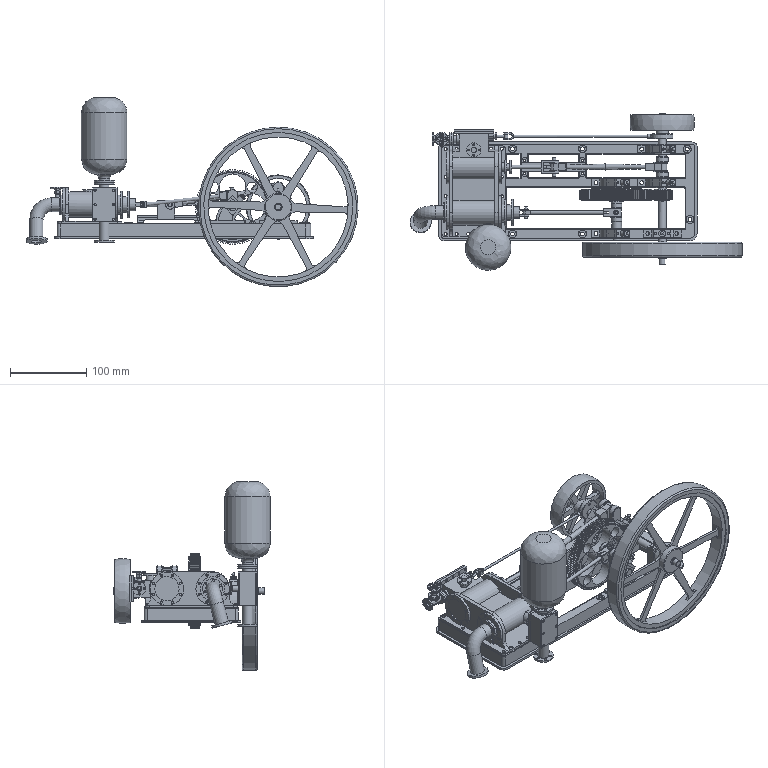Assembly | NX | mm | 86 component files | 86 solids | 2631 faces | box 436.98 x 206 x 248.97 mm | volume 711241 mm3 | cylinder 1021 | plane 907 | other 480 | spline 134 | torus 66 | cone 18 | sphere 5 | commonest cylinder face diameters 3 x200 2 x150 93.5 x96 5 x87 4 x55 2.5 x51 10 x47 6 x39
Bill of materials:
unnamed part 1 | 1 |  | Long slender cylindrical pin with a countersunk-style conical head, a short larger-diameter shoulder section below the head, then a long smaller-diameter plain shank ending in a flat end.
unnamed part 2 | 1 |  | Clevis/fork block: rectangular solid body with a rectangular slot open at one end, forming two parallel lugs with rounded ends and aligned through-holes; a smaller through-hole passes through the body at the base of the slot.
unnamed part 3 | 1 |  | Stepped annular flange body: a larger-diameter disc and a smaller-diameter disc joined by a cylindrical hub, all sharing a large central bore; both discs have rings of axial bolt holes (8 visible in face view).
unnamed part 4 | 1 |  | Hollow cylindrical tube, open at one end, with the other end closed by a rounded/conical taper ending in a short small-diameter neck with a central through-hole.
unnamed part 5 | 1 |  | Plain flat annular ring (washer- or spacer-like) with a centred circular through-hole and moderate thickness.
unnamed part 6 | 1 |  | Thick cylindrical sleeve/bushing with a large concentric through-bore and a relatively thin wall compared with the similar ring part.
unnamed part 7 | 1 |  | Long round rod with a rounded eye end at one end (transverse through-hole) and a square block at the other end with a small square hole and a slot.
unnamed part 8 | 1 |  | Very long slender round rod with a small clevis fork at one end: two parallel lugs with aligned cross-holes; the opposite end is plain.
unnamed part 9 | 5 |  | Rectangular flat plate (block) with one large central through-hole and two smaller through-holes, one near each end, all in a line along the long axis.
unnamed part 10 | 4 |  | Angled bracket: a flat base strip with a through-hole at each end, and a raised web rising at about 45 degrees into a U-shaped fork with two parallel tabs, each with a through-hole; fillets blend the web into the base.
unnamed part 11 | 1 |  | Housing/frame: a rectangular base plate with perimeter holes, two upright end plates with rounded tops, each with two large bores and surrounding small hole patterns, joined by two parallel cylindrical shells; a small cylindrical boss with a bore projects from one shell near one end plate.
unnamed part 12 | 1 |  | Flanged tee-shaped body: a barrel-shaped, bulging central body with a circular flange at each end and a third circular flange on a short branch on top; each flange has four bolt holes and a central bore.
unnamed part 13 | 1 |  | Short hollow cylinder with one step: a wider ring section at one end and a slightly smaller-diameter section at the other, with a plain through bore. Looks like a flanged bushing or sleeve.
unnamed part 14 | 1 |  | Bracket with a flat rectangular base plate and two parallel rectangular uprights, forming a U-shaped fork in the front profile. The base has one through hole at each end, each upright has a small hole in its top face, and there are fillets where the uprights meet the base.
unnamed part 15 | 1 |  | Thin-walled circular ring or band with one short solid cylindrical stub sticking out radially from its outer surface. The stub has a small fillet where it joins the ring.
unnamed part 16 | 1 |  | Long, slender cylindrical rod. At one end it joins, at right angles, a short hollow cylindrical boss or eye with a through bore, whose axis is perpendicular to the rod.
unnamed part 17 | 1 |  | Thin flat ring with a small step: a slightly larger outer diameter on one face and a slightly smaller one on the other. It has a large central bore relative to its outer diameter.
unnamed part 18 | 1 |  | Straight-tooth spur gear with about 24 external teeth, a central through bore with a single rectangular keyway, and a raised hub face or shoulder on each side.
unnamed part 19 | 1 |  | Solid stepped cylindrical pin or shaft: a larger-diameter central body with smaller-diameter coaxial journals at both ends.
unnamed part 20 | 1 |  | Prismatic block with angled (chamfered) faces on one side and a rounded-end U-slot cut in from that side. It has a stepped profile (a narrower raised portion on a wider base) and a rectangular recess or pocket visible in one face of the isometric view.
unnamed part 21 | 1 |  | Block with a through bore. In the end profile one side is a rounded semicircle and the other side tapers to flat faces, giving a teardrop or D shape. Thin raised lips or flanges at both axial ends border a slightly recessed middle band.
unnamed part 22 | 1 |  | Spoked wheel with six straight spokes joining a central hub to an outer rim. The hub has a small central through hole and the rim has a slightly crowned outer surface.
unnamed part 23 | 1 |  | Thin circular disc with rounded edges, pierced by four large circular holes evenly spaced around a smaller central hole.
unnamed part 24 | 5 |  | Ball stud: a spherical ball on a short narrowed neck, standing on a cylindrical disc base. The base appears stepped, with a smaller-diameter boss or section on the side opposite the ball.
unnamed part 25 | 1 |  | Flanged cylindrical bushing: a short cylindrical shank joined to a larger-diameter cylindrical flange, with a plain through bore on the common axis.
unnamed part 26 | 1 |  | Thin-walled plain ring: short hollow cylinder with a large bore and a narrow radial wall.
unnamed part 27 | 1 |  | Grooved disc/pulley-like wheel: solid cylindrical disc with one rectangular circumferential groove at mid-width and a small central through bore.
unnamed part 28 | 1 |  | Spur gear with straight external teeth and a web pierced by lightening holes: four large and four small circular cutouts arranged around a central bore that has a keyway notch.
unnamed part 29 | 1 |  | Plain flat ring/washer-like annulus with a moderate radial wall, thicker relative to its diameter than the other thin ring.
unnamed part 30 | 1 |  | Stepped solid cylindrical shaft/pin: a longer central section of larger diameter with a shorter, smaller-diameter journal at each end.
unnamed part 31 | 1 |  | Thin flat circular disc/washer with a small central through hole.
unnamed part 32 | 1 |  | Flanged hub/flange mount: a round flange with four through holes on a bolt circle, a coaxial cylindrical boss on one side, and a central through bore.
unnamed part 33 | 1 |  | Elongated mounting bracket/strap: a long rectangular bar with a T-shaped end profile, supported at each end by filleted posts down to flat foot lugs. Each end has two rounded-end tabs, each with a through hole (four holes in total).
unnamed part 34 | 1 |  | Clamp/bearing-block-like body: a block with one flat, slightly tapered mounting side and one semicircular rounded side. It has a large through bore, a raised lip or rim at each axial end, and a small radial hole through the top into the bore.
unnamed part 35 | 1 |  | Flat rectangular plate with six round through holes, three evenly spaced along each long edge.
unnamed part 36 | 1 |  | Stepped solid cylindrical shaft with four coaxial diameters that get smaller from a large base section to a slender tip section.
unnamed part 37 | 1 |  | Single-throw crank-shaped shaft: two coaxial cylindrical end shafts joined by two parallel obround webs and an offset cylindrical pin between them.
unnamed part 38 | 1 |  | Circular flat flange plate with a raised cylindrical hub in the center, a central through bore, and four through holes evenly spaced on a bolt circle.
unnamed part 39 | 5 |  | Square block with rounded corners and a large round through bore along its axis. Square end flanges stand slightly proud of an inset middle body.
unnamed part 40 | 1 |  | Round drum with a rim flange at each end, forming a shallow groove between them, plus a smaller cylindrical hub on one side. The hub's through bore is off-center from the drum, and a small through hole sits on the opposite side of the face.
unnamed part 41 | 1 |  | Flat circular flange ring with a central bore, eight through holes evenly spaced on a bolt circle, and a raised annular face around the bore.
unnamed part 42 | 1 |  | Hexagonal prism with a plain cylindrical through hole in the center.
unnamed part 43 | 1 |  | 90-degree bent tube with a flange at each end. One flange has six bolt holes; the other is a plain annular flange with no visible holes.
unnamed part 44 | 1 |  | D-shaped block, rounded at one end and flat at the other, with a large round through bore. Thin lips at both ends stand slightly proud of the middle body.
unnamed part 45 | 1 |  | Flanged bushing: a circular flange with four bolt holes, a cylindrical shank on one side, and a central through bore.
unnamed part 46 | 1 |  | Plain flat annular ring (washer shape) with a central round hole.
unnamed part 47 | 1 |  | Short tubular neck joined to a circular flange with six evenly spaced bolt holes and a central through bore.
unnamed part 48 | 1 |  | Solid circular disc (blind-flange shape) with eight evenly spaced bolt holes and a raised circular face on one side; there is no central bore.
unnamed part 49 | 1 |  | Flanged cylindrical hub: a circular flange with four through holes, a cylindrical hub with a raised collar ring partway along it, and a central through bore.
unnamed part 50 | 1 |  | Solid rectangular block with one cylindrical through hole passing straight through between two opposite faces.
unnamed part 51 | 5 |  | Short hollow cylindrical sleeve (bushing-like tube) with a stepped outer diameter: a reduced-diameter band at one end.
unnamed part 52 | 1 |  | Slender rod with a square block at each end. The faceted shaft tapers from a thicker middle toward both ends.
unnamed part 53 | 1 |  | Vertical housing made of a rectangular box with open, bolt-holed rims on two sides, plus pipe stubs ending in circular bolted flanges top and bottom.
unnamed part 54 | 1 |  | Rectangular mounting plate with six perimeter holes and a central hole. A cylindrical pipe stub projects perpendicular from one face and ends in a circular flange.
unnamed part 55 | 1 |  | Diamond-shaped (two-lobe) flange with rounded ends, a hole in each lobe, a larger central through hole, and a cylindrical boss on one side.
unnamed part 56 | 1 |  | Thin strip bent into a U (hairpin) shape. Each leg has a slot open at its end, and a short hollow cylindrical boss stands on the outer face near the bend.
unnamed part 57 | 1 |  | Long straight round pin/shaft with a reduced-diameter step at each end.
unnamed part 58 | 1 |  | Box-like bracket with a channel-shaped body, two round-ended lugs with coaxial through holes, an elongated slot in one face, a hole in another face, and hooked/stepped feet at the bottom.
unnamed part 59 | 1 |  | Long rectangular frame plate with rounded corners, divided by webs into six rectangular through openings. It has many small holes around the perimeter and on the webs, several raised or counterbored hole bosses, and a stepped lip around the base.
unnamed part 60 | 1 |  | Spoked wheel: a circular rim joined by six straight spokes to a central hub with a small central bore.
unnamed part 61 | 1 |  | Round flange part: a large flat circular disc with a ring of 8 through-holes near its edge and a central bore. A short shallow raised step is on one face. On the other face, a cylindrical neck sticks out and ends in a smaller circular flange with its own ring of small holes around the central bore.
unnamed part 62 | 1 |  | Cup-shaped wheel: a thin-walled cylindrical rim with two grooves running around its outside. A web sits inside the rim, recessed from one face, with a central hole and six large round lightening holes evenly spaced around it.
unnamed part 63 | 1 |  | Plain flat ring (annulus) with a large central through-hole and parallel flat faces, shaped like a washer.
unnamed part 64 | 1 |  | Capsule-shaped closed body: a cylinder with rounded, dome-like ends. At one end, a short narrow neck flares into a small circular flange with several small holes.
unnamed part 65 | 1 |  | Machined block bracket: a flat rectangular mounting plate with two rows of 5 through-holes, joined at a right angle to a block-shaped body. The body has a flat top with a counterbored hole, ledges/rails along its long sides, a concave curved cutout at the end away from the plate, elongated slots through the body, and a boss with a bore and small holes next to the plate.
unnamed part 66 | 1 |  | Single-throw crank-type shaft: a long stepped cylindrical shaft with two parallel obround (rounded-end) webs near one end, joined by an offset cylindrical pin. Several short diameter steps run along the shaft, with shallow slot-like features that may be keyways.
unnamed part 67 | 1 |  | Flat rectangular plate of constant thickness with 14 round through-holes spaced along its edges: 5 along each long edge (including the corners) and 2 more along each short edge.
Mates:
1. fix | base 1 component
2. concentric | base 1 edge | support_stand 1 edge
3. parallel | support_stand 1 face | base 1 face
4. concentric | base 1 edge | inclined_frame 4 arc
5. parallel | inclined_frame 4 face | base 1 face
6. concentric | inclined_frame 4 edge | inclined_frame_top_plate 5 arc
7. parallel | inclined_frame_top_plate 5 face | inclined_frame 4 face
8. center | inclined_frame 4 face | inclined_frame 4 face | filler_block 5 face | filler_block 5 face
9. center | filler_block 5 face | filler_block 5 face | inclined_frame 4 face | inclined_frame 4 face
10. touch align | filler_block 5 face | inclined_frame 4 face
11. concentric | base 1 edge | inclined_frame 3 arc
12. parallel | inclined_frame 3 face | base 1 face
13. concentric | base 1 edge | inclined_frame 2 arc
14. parallel | inclined_frame 2 face | base 1 face
15. concentric | base 1 edge | inclined_frame 1 arc
16. parallel | inclined_frame 1 face | base 1 face
17. concentric | inclined_frame 3 edge | inclined_frame_top_plate 4 arc
18. parallel | inclined_frame_top_plate 4 face | inclined_frame 3 face
19. concentric | inclined_frame 2 edge | inclined_frame_top_plate 3 arc
20. parallel | inclined_frame_top_plate 3 face | inclined_frame 2 face
21. concentric | inclined_frame 1 edge | inclined_frame_top_plate 2 arc
22. parallel | inclined_frame_top_plate 2 face | inclined_frame 1 face
23. center | filler_block 4 face | filler_block 4 face | inclined_frame 3 face | inclined_frame 3 face
24. center | filler_block 4 face | filler_block 4 face | inclined_frame 3 face | inclined_frame 3 face
25. touch align | filler_block 4 face | inclined_frame_top_plate 4 face
26. center | filler_block 3 face | filler_block 3 face | inclined_frame 2 face | inclined_frame_top_plate 3 face
27. center | filler_block 3 face | filler_block 3 face | inclined_frame 2 face | inclined_frame 2 face
28. touch align | filler_block 3 face | inclined_frame 2 face
29. center | filler_block 2 face | filler_block 2 face | inclined_frame 1 face | inclined_frame_top_plate 2 face
30. center | filler_block 2 face | filler_block 2 face | inclined_frame 1 face | inclined_frame 1 face
31. touch align | filler_block 2 face | inclined_frame 1 face
32. touch align | base 1 face | piston_cyl_body 1 face
33. center | piston_cyl_body 1 face | piston_cyl_body 1 face | base 1 face | base 1 face
34. touch align | piston_cyl_body 1 face | ext_cylinder_body 1 face
35. center | ext_cylinder_body 1 face | ext_cylinder_body 1 face | piston_cyl_body 1 face | piston_cyl_body 1 face
36. concentric | ext_cylinder_body 1 edge | ext_end_plate 1 arc
37. parallel | ext_end_plate 1 face | ext_cylinder_body 1 face
38. concentric | piston_cyl_body 1 edge | air_cylinder_conn_plate 1 arc
39. parallel | air_cylinder_conn_plate 1 face | base 1 face
40. concentric | air_cylinder_conn_plate 1 edge | water_tank_cyl_body 1 edge
41. parallel | water_tank_cyl_body 1 face | air_cylinder_conn_plate 1 face
42. concentric | water_cyl_tank_end_plate 1 arc | water_tank_cyl_body 1 edge
43. parallel | water_cyl_tank_end_plate 1 face | water_tank_cyl_body 1 face
44. concentric | water_tank_cyl_body 1 edge | water_chamber 1 arc
45. concentric | water_chamber 1 edge | water_tank_cyl_body 1 edge
46. touch align | crankshaft 1 face | filler_block 2 face
47. center | crankshaft 1 face | crankshaft 1 face | piston_cyl_body 1 face
48. touch align | filler_block 1 face | crankshaft 1 face
49. center | filler_block 1 face | filler_block 1 face | base 1 face | base 1 face
50. parallel | filler_block 1 face | base 1 face
51. touch align | filler_block 1 face | inclined_frame_top_plate 1 face
52. center | inclined_frame_top_plate 1 face | inclined_frame_top_plate 1 face | filler_block 1 face | filler_block 1 face
53. concentric | upright_frame 1 arc | inclined_frame_top_plate 1 edge
54. parallel | upright_frame 1 face | inclined_frame_top_plate 1 face
55. touch align | big_flywheel 1 face | crankshaft 1 face
56. distance | big_flywheel 1 face | base 1 face
57. touch align | small_gear 1 face | crankshaft 1 face
58. touch align | crankshaft_2 1 face | filler_block 5 face
59. center | crankshaft_2 1 face | crankshaft_2 1 face | piston_cyl_body 1 face
60. touch align | big_gear 1 face | crankshaft_2 1 face
61. parallel | crankshaft_2 1 face | big_gear 1 face
62. center | big_gear 1 face | big_gear 1 face | filler_block 4 face | crankshaft_2 1 face
63. center | small_gear 1 face | small_gear 1 face | big_gear 1 face | big_gear 1 face
64. concentric | washer 1 arc | big_gear 1 edge
65. touch align | link_1 1 face | big_conn_block 1 face
66. center | link_1 1 face | link_1 1 face | big_conn_block 1 face | big_conn_block 1 face
67. center | link_1 1 face | link_1 1 face | big_conn_block 1 face | big_conn_block 1 face
68. touch align | link_1 1 face | small_conn_block 1 face
69. center | small_conn_block 1 face | small_conn_block 1 face | link_1 1 face | link_1 1 face
70. center | small_conn_block 1 face | small_conn_block 1 face | link_1 1 face | link_1 1 face
71. touch align | big_conn_block 1 face | crankshaft 1 face
72. center | big_conn_block 1 face | big_conn_block 1 face | piston_cyl_body 1 face
73. concentric | piston_ring 1 arc | piston 1 edge
74. concentric | link_2 1 edge | piston 1 arc
75. touch align | link_2 1 face | piston_cyl_body 1 face
76. distance | piston_cyl_body 1 face | base 1 face
77. concentric | link_slider 1 arc | link_2 1 edge
78. touch align | small_conn_block 1 face | link_slider 1 face
79. touch align | link_pin 1 face | link_slider 1 face
80. center | link_pin 1 face | link_pin 1 face | link_slider 1 face | link_slider 1 face
81. center | link_3_large_block 1 face | link_3_large_block 1 face | link_3 1 face | link_3 1 face
82. touch align | link_3_large_block 1 face | link_3 1 face
83. center | link_3_large_block 1 face | link_3_large_block 1 face | link_3 1 face | link_3 1 face
84. touch align | link_3_large_block 1 face | crankshaft_2 1 face
85. center | link_3_large_block 1 face | link_3_large_block 1 face | crankshaft_2 1 face | crankshaft_2 1 face
86. concentric | link_3_large_ring 1 edge | link_3_large_block 1 edge
87. parallel | link_3 1 face | link_3_large_ring 1 face
88. concentric | round_plate 1 edge | link_4 1 edge
89. concentric | int_pipe_flywheel 1 edge | round_plate 1 arc
90. concentric | lumen 1 arc | int_pipe_flywheel 1 arc
91. concentric | link_4_block 1 edge | link_4 1 edge
92. touch align | link_4_block 1 face | link_3 1 face
93. center | link_4_block 1 face | link_4_block 1 face | link_3 1 face | link_3 1 face
94. touch align | lumen 1 face | piston_cyl_body 1 face
95. touch align | link_4_pin 1 face | link_4_block 1 face
96. center | link_4_pin 1 face | link_4_pin 1 face | link_4_block 1 face | link_4_block 1 face
97. concentric | link_5 1 arc | link_5_ring 1 edge
98. parallel | link_5 1 face | link_5_ring 1 face
99. touch align | eccentric_cam 1 face | link_5_ring 1 face
100. center | eccentric_cam 1 face | eccentric_cam 1 face | link_5_ring 1 face | link_5_ring 1 face
101. touch align | eccentric_cam 1 face | crankshaft 1 face
102. center | eccentric_cam 1 face | eccentric_cam 1 face | ext_cylinder_body 1 face
103. touch align | link_6 1 face | link_5 1 face
104. center | link_5 1 face | link_5 1 face | link_6 1 face | link_6 1 face
105. touch align | link_6 1 face | ext_cylinder_body 1 face
106. concentric | piston_cyl_body 1 edge | end_cover_1 1 edge
107. concentric | piston_cyl_body 1 edge | end_cover_1 1 edge
108. concentric | piston_cyl_body 1 edge | end_cap_2 1 edge
109. concentric | end_cap_2 1 edge | piston_cyl_body 1 edge
110. concentric | end_cap_2 1 edge | ext_conn_pipe 1 arc
111. concentric | ext_conn_pipe 1 arc | end_cap_2 1 edge
112. concentric | piston_cyl_body 1 edge | end_cap_3 1 edge
113. concentric | end_cap_3 1 edge | piston_cyl_body 1 edge
114. concentric | end_cap_3_bushing 1 edge | end_cap_3 1 edge
115. concentric | end_cap_3_washer 1 arc | end_cap_3_bushing 1 arc
116. concentric | end_cap_3_outer_cap 1 edge | end_cap_3_washer 1 edge
117. distance | end_cap_3_outer_cap 1 face | end_cap_3 1 face
118. concentric | piston_cyl_body 1 edge | end_cap_4 1 edge
119. concentric | end_cap_4 1 edge | piston_cyl_body 1 edge
120. concentric | end_cap_4_bushing 1 edge | end_cap_4 1 edge
121. concentric | end_cap_4_washer 1 arc | end_cap_4_bushing 1 edge
122. concentric | end_cap_4_outer_cap 1 edge | end_cap_4_washer 1 edge
123. touch align | end_cap_4_outer_cap 1 face | end_cap_4 1 face
124. concentric | ext_cylinder_body 1 edge | ext_cylinder_end_cover 1 edge
125. concentric | ext_cylinder_conn_end_cover 1 edge | ext_cylinder_body 1 edge
126. concentric | ext_cylinder_conn_end_cover 1 edge | ext_pipe 1 arc
127. parallel | ext_pipe 1 face | ext_cylinder_body 1 face
128. concentric | ext_pipe 1 edge | ext_pipe_upper_end_cover 1 edge
129. concentric | ext_pipe_upper_end_cover 1 edge | ext_pipe 1 edge
130. concentric | ext_pipe 1 edge | ext_cylinder_conn_end_cover 1 edge
131. parallel | ext_cylinder_body 1 face | piston_cyl_body 1 face
132. touch align | valve_core 1 face | ext_pipe_upper_end_cover 1 face
133. distance | valve_core 1 face | ext_pipe_upper_end_cover 1 face
134. concentric | ext_pipe_gasket 1 arc | ext_pipe_upper_end_cover 1 edge
135. concentric | ext_pipe_conn_block 1 arc | ext_pipe_gasket 1 edge
136. concentric | rotary_switch 1 arc | valve_core 1 edge
137. concentric | vent_pipe_cap 5 edge | inclined_frame_top_plate 5 edge
138. concentric | vent_end_cap 5 edge | vent_pipe_cap 5 arc
139. concentric | inclined_frame_top_plate 4 edge | vent_pipe_cap 4 edge
140. concentric | vent_end_cap 4 edge | vent_pipe_cap 4 arc
141. concentric | inclined_frame_top_plate 1 edge | vent_pipe_cap 3 edge
142. concentric | vent_end_cap 3 edge | vent_pipe_cap 3 arc
143. concentric | vent_pipe_cap 2 edge | inclined_frame_top_plate 3 edge
144. concentric | vent_pipe_cap 1 edge | inclined_frame_top_plate 2 edge
145. concentric | vent_end_cap 2 edge | vent_pipe_cap 2 arc
146. concentric | vent_end_cap 1 edge | vent_pipe_cap 1 arc
147. concentric | ext_cylinder_body_shaft_sleeve 1 edge | ext_cylinder_body 1 edge
148. concentric | ext_cylinder_body_washer 1 arc | ext_cylinder_body_shaft_sleeve 1 arc
149. concentric | ext_cylinder_body_end_cover 1 edge | ext_cylinder_body 1 edge
150. touch align | ext_cylinder_body_end_cover 1 face | ext_cylinder_body 1 face